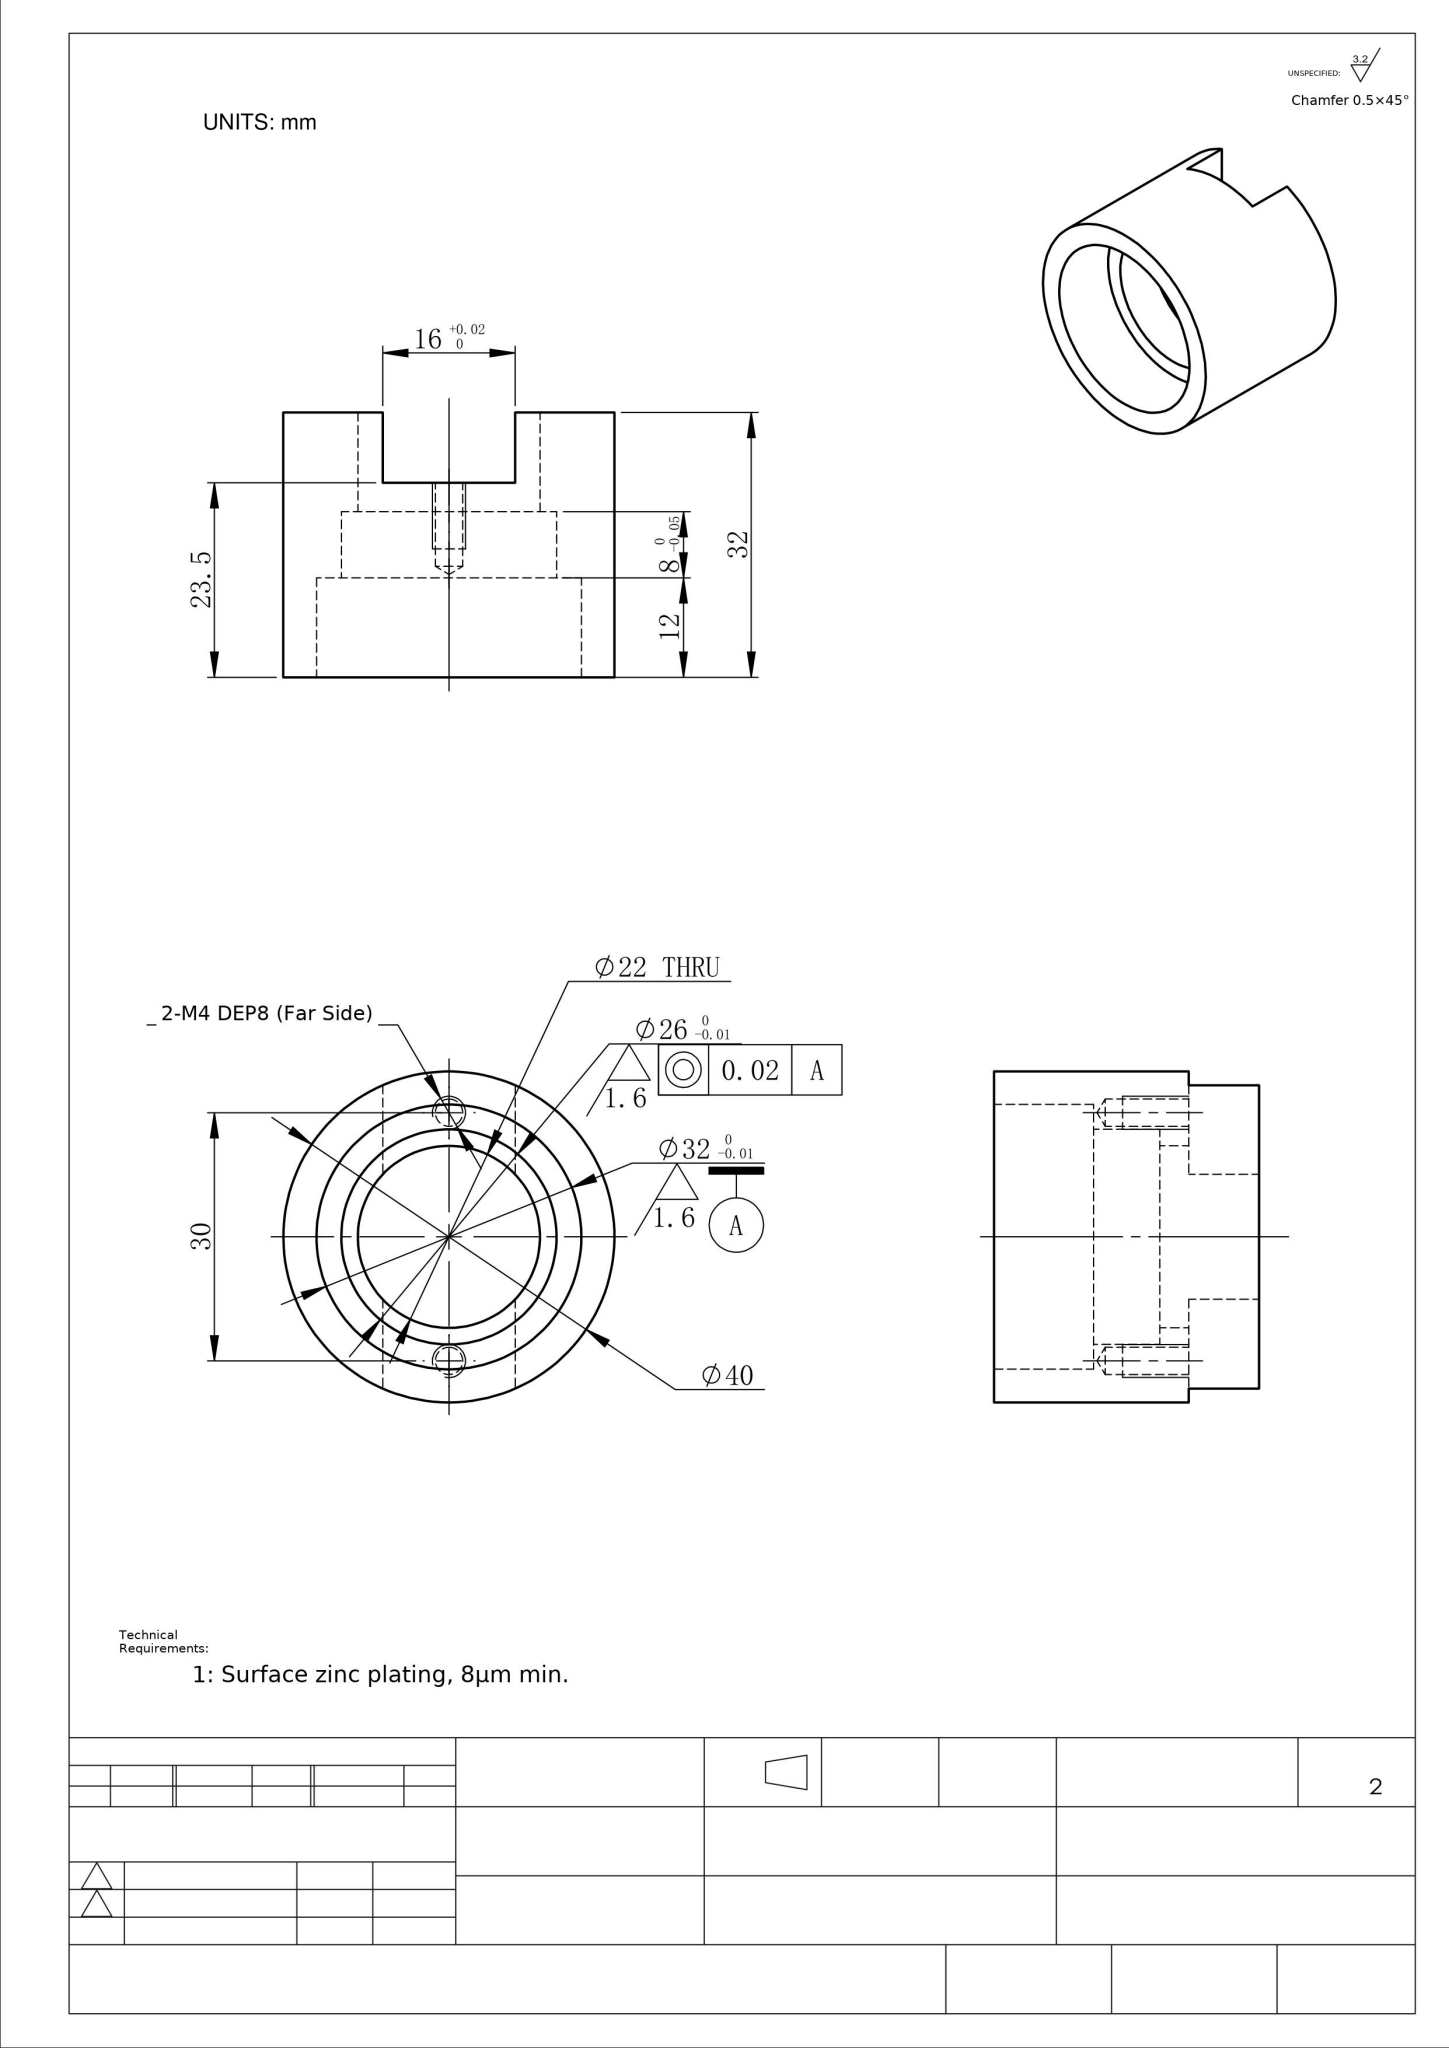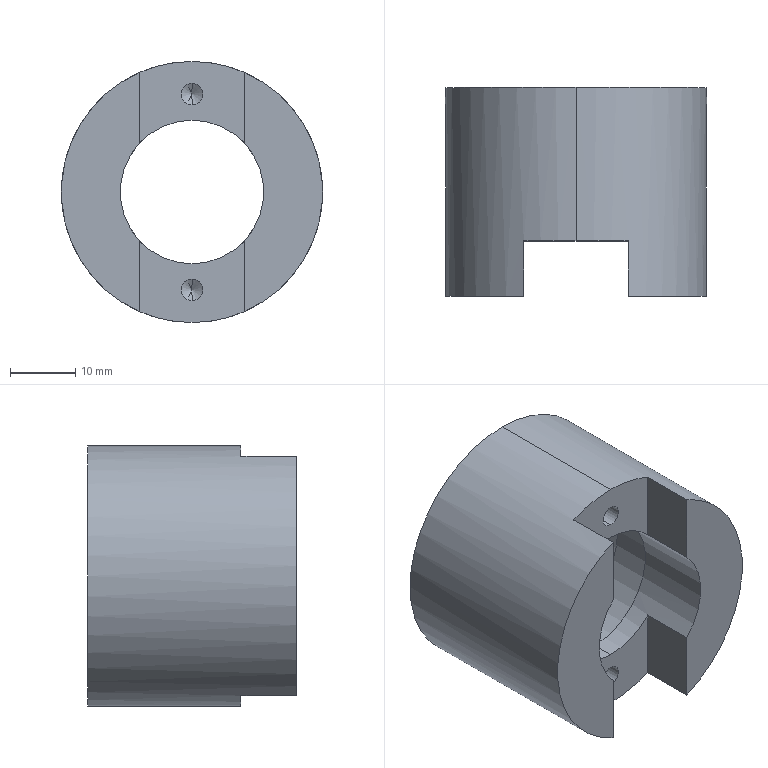Part | NX | mm | 1 solid | 27 faces | box 40 x 32 x 40 mm | volume 18985 mm3 | cylinder 12 | plane 11 | cone 4 | commonest cylinder face diameters 3.3 x4 22 x2 26 x2 32 x2 40 x2
STEP:
#1=COLOUR_RGB('',0.7961,0.8235,0.9373);
#2=FILL_AREA_STYLE_COLOUR('',#1);
#3=FILL_AREA_STYLE('',(#2));
#4=SURFACE_STYLE_FILL_AREA(#3);
#5=SURFACE_SIDE_STYLE('',(#4));
#6=SURFACE_STYLE_USAGE(.BOTH.,#5);
#7=PRESENTATION_STYLE_ASSIGNMENT((#6));
#8=CARTESIAN_POINT('',(0.,18.6,16.65));
#9=VERTEX_POINT('',#8);
#10=CARTESIAN_POINT('',(0.,18.6,13.35));
#11=VERTEX_POINT('',#10);
#12=CARTESIAN_POINT('',(0.,18.6,15.));
#13=DIRECTION('',(0.,-1.,0.));
#14=DIRECTION('',(0.,0.,-1.));
#15=AXIS2_PLACEMENT_3D('',#12,#13,#14);
#16=CIRCLE('',#15,1.65);
#17=EDGE_CURVE('',#9,#11,#16,.T.);
#18=ORIENTED_EDGE('',*,*,#17,.F.);
#19=CARTESIAN_POINT('',(0.,8.5,16.65));
#20=VERTEX_POINT('',#19);
#21=CARTESIAN_POINT('',(0.,8.5,16.65));
#22=DIRECTION('',(0.,-1.,0.));
#23=VECTOR('',#22,1000.);
#24=LINE('',#21,#23);
#25=EDGE_CURVE('',#9,#20,#24,.T.);
#26=ORIENTED_EDGE('',*,*,#25,.T.);
#27=CARTESIAN_POINT('',(0.,8.5,13.35));
#28=VERTEX_POINT('',#27);
#29=CARTESIAN_POINT('',(0.,8.5,15.));
#30=DIRECTION('',(0.,-1.,0.));
#31=DIRECTION('',(0.,0.,-1.));
#32=AXIS2_PLACEMENT_3D('',#29,#30,#31);
#33=CIRCLE('',#32,1.65);
#34=EDGE_CURVE('',#20,#28,#33,.T.);
#35=ORIENTED_EDGE('',*,*,#34,.T.);
#36=CARTESIAN_POINT('',(0.,8.5,13.35));
#37=DIRECTION('',(0.,-1.,0.));
#38=VECTOR('',#37,1000.);
#39=LINE('',#36,#38);
#40=EDGE_CURVE('',#11,#28,#39,.T.);
#41=ORIENTED_EDGE('',*,*,#40,.F.);
#42=EDGE_LOOP('',(#18,#26,#35,#41));
#43=FACE_OUTER_BOUND('',#42,.T.);
#44=CARTESIAN_POINT('',(0.,8.5,15.));
#45=DIRECTION('',(0.,-1.,0.));
#46=DIRECTION('',(0.,0.,-1.));
#47=AXIS2_PLACEMENT_3D('',#44,#45,#46);
#48=CYLINDRICAL_SURFACE('',#47,1.65);
#49=ADVANCED_FACE('',(#43),#48,.F.);
#50=STYLED_ITEM('',(#7),#49);
#51=(LENGTH_UNIT()NAMED_UNIT(*)SI_UNIT(.MILLI.,.METRE.));
#52=UNCERTAINTY_MEASURE_WITH_UNIT(LENGTH_MEASURE(0.00001),#51,'','');
#53=(NAMED_UNIT(*)PLANE_ANGLE_UNIT()SI_UNIT($,.RADIAN.));
#54=(NAMED_UNIT(*)SI_UNIT($,.STERADIAN.)SOLID_ANGLE_UNIT());
#55=(GEOMETRIC_REPRESENTATION_CONTEXT(3)GLOBAL_UNCERTAINTY_ASSIGNED_CONTEXT((#52))GLOBAL_UNIT_ASSIGNED_CONTEXT((#51,#53,#54))REPRESENTATION_CONTEXT('',''));
#56=MECHANICAL_DESIGN_GEOMETRIC_PRESENTATION_REPRESENTATION('',(#50),#55);
#57=COLOUR_RGB('',0.7961,0.8235,0.9373);
#58=FILL_AREA_STYLE_COLOUR('',#57);
#59=FILL_AREA_STYLE('',(#58));
#60=SURFACE_STYLE_FILL_AREA(#59);
#61=SURFACE_SIDE_STYLE('',(#60));
#62=SURFACE_STYLE_USAGE(.BOTH.,#61);
#63=PRESENTATION_STYLE_ASSIGNMENT((#62));
#64=CARTESIAN_POINT('',(-0.,19.591,15.));
#65=VERTEX_POINT('',#64);
#66=CARTESIAN_POINT('',(0.,18.6,13.35));
#67=DIRECTION('',(0.,-0.515,-0.8572));
#68=VECTOR('',#67,1000.);
#69=LINE('',#66,#68);
#70=EDGE_CURVE('',#65,#11,#69,.T.);
#71=ORIENTED_EDGE('',*,*,#70,.F.);
#72=CARTESIAN_POINT('',(0.,18.6,16.65));
#73=DIRECTION('',(0.,-0.515,0.8572));
#74=VECTOR('',#73,1000.);
#75=LINE('',#72,#74);
#76=EDGE_CURVE('',#65,#9,#75,.T.);
#77=ORIENTED_EDGE('',*,*,#76,.T.);
#78=ORIENTED_EDGE('',*,*,#17,.T.);
#79=EDGE_LOOP('',(#71,#77,#78));
#80=FACE_OUTER_BOUND('',#79,.T.);
#81=CARTESIAN_POINT('',(0.,18.6,15.));
#82=DIRECTION('',(0.,-1.,0.));
#83=DIRECTION('',(0.,0.,-1.));
#84=AXIS2_PLACEMENT_3D('',#81,#82,#83);
#85=CONICAL_SURFACE('',#84,1.65,1.03);
#86=ADVANCED_FACE('',(#80),#85,.F.);
#87=CARTESIAN_POINT('',(-0.,19.591,-15.));
#88=VERTEX_POINT('',#87);
#89=CARTESIAN_POINT('',(0.,18.6,-16.65));
#90=VERTEX_POINT('',#89);
#91=CARTESIAN_POINT('',(0.,18.6,-16.65));
#92=DIRECTION('',(0.,-0.515,-0.8572));
#93=VECTOR('',#92,1000.);
#94=LINE('',#91,#93);
#95=EDGE_CURVE('',#88,#90,#94,.T.);
#96=ORIENTED_EDGE('',*,*,#95,.F.);
#97=CARTESIAN_POINT('',(0.,18.6,-13.35));
#98=VERTEX_POINT('',#97);
#99=CARTESIAN_POINT('',(0.,18.6,-13.35));
#100=DIRECTION('',(0.,-0.515,0.8572));
#101=VECTOR('',#100,1000.);
#102=LINE('',#99,#101);
#103=EDGE_CURVE('',#88,#98,#102,.T.);
#104=ORIENTED_EDGE('',*,*,#103,.T.);
#105=CARTESIAN_POINT('',(0.,18.6,-15.));
#106=DIRECTION('',(0.,-1.,0.));
#107=DIRECTION('',(0.,0.,-1.));
#108=AXIS2_PLACEMENT_3D('',#105,#106,#107);
#109=CIRCLE('',#108,1.65);
#110=EDGE_CURVE('',#98,#90,#109,.T.);
#111=ORIENTED_EDGE('',*,*,#110,.T.);
#112=EDGE_LOOP('',(#96,#104,#111));
#113=FACE_OUTER_BOUND('',#112,.T.);
#114=CARTESIAN_POINT('',(0.,18.6,-15.));
#115=DIRECTION('',(0.,-1.,0.));
#116=DIRECTION('',(0.,0.,-1.));
#117=AXIS2_PLACEMENT_3D('',#114,#115,#116);
#118=CONICAL_SURFACE('',#117,1.65,1.03);
#119=ADVANCED_FACE('',(#113),#118,.F.);
#120=ORIENTED_EDGE('',*,*,#110,.F.);
#121=CARTESIAN_POINT('',(0.,8.5,-13.35));
#122=VERTEX_POINT('',#121);
#123=CARTESIAN_POINT('',(0.,8.5,-13.35));
#124=DIRECTION('',(0.,-1.,0.));
#125=VECTOR('',#124,1000.);
#126=LINE('',#123,#125);
#127=EDGE_CURVE('',#98,#122,#126,.T.);
#128=ORIENTED_EDGE('',*,*,#127,.T.);
#129=CARTESIAN_POINT('',(0.,8.5,-16.65));
#130=VERTEX_POINT('',#129);
#131=CARTESIAN_POINT('',(0.,8.5,-15.));
#132=DIRECTION('',(0.,-1.,0.));
#133=DIRECTION('',(0.,0.,-1.));
#134=AXIS2_PLACEMENT_3D('',#131,#132,#133);
#135=CIRCLE('',#134,1.65);
#136=EDGE_CURVE('',#122,#130,#135,.T.);
#137=ORIENTED_EDGE('',*,*,#136,.T.);
#138=CARTESIAN_POINT('',(0.,8.5,-16.65));
#139=DIRECTION('',(0.,-1.,0.));
#140=VECTOR('',#139,1000.);
#141=LINE('',#138,#140);
#142=EDGE_CURVE('',#90,#130,#141,.T.);
#143=ORIENTED_EDGE('',*,*,#142,.F.);
#144=EDGE_LOOP('',(#120,#128,#137,#143));
#145=FACE_OUTER_BOUND('',#144,.T.);
#146=CARTESIAN_POINT('',(0.,8.5,-15.));
#147=DIRECTION('',(0.,-1.,0.));
#148=DIRECTION('',(0.,0.,-1.));
#149=AXIS2_PLACEMENT_3D('',#146,#147,#148);
#150=CYLINDRICAL_SURFACE('',#149,1.65);
#151=ADVANCED_FACE('',(#145),#150,.F.);
#152=CARTESIAN_POINT('',(-8.,8.5,-7.55));
#153=VERTEX_POINT('',#152);
#154=CARTESIAN_POINT('',(0.,8.5,-11.));
#155=VERTEX_POINT('',#154);
#156=CARTESIAN_POINT('',(0.,8.5,0.));
#157=DIRECTION('',(0.,-1.,0.));
#158=DIRECTION('',(0.,0.,1.));
#159=AXIS2_PLACEMENT_3D('',#156,#157,#158);
#160=CIRCLE('',#159,11.);
#161=EDGE_CURVE('',#153,#155,#160,.T.);
#162=ORIENTED_EDGE('',*,*,#161,.T.);
#163=CARTESIAN_POINT('',(0.,12.,-11.));
#164=VERTEX_POINT('',#163);
#165=CARTESIAN_POINT('',(0.,88.583,-11.));
#166=DIRECTION('',(0.,1.,0.));
#167=VECTOR('',#166,1000.);
#168=LINE('',#165,#167);
#169=EDGE_CURVE('',#155,#164,#168,.T.);
#170=ORIENTED_EDGE('',*,*,#169,.T.);
#171=CARTESIAN_POINT('',(0.,12.,11.));
#172=VERTEX_POINT('',#171);
#173=CARTESIAN_POINT('',(0.,12.,0.));
#174=DIRECTION('',(0.,1.,0.));
#175=DIRECTION('',(0.,0.,1.));
#176=AXIS2_PLACEMENT_3D('',#173,#174,#175);
#177=CIRCLE('',#176,11.);
#178=EDGE_CURVE('',#164,#172,#177,.T.);
#179=ORIENTED_EDGE('',*,*,#178,.T.);
#180=CARTESIAN_POINT('',(0.,8.5,11.));
#181=VERTEX_POINT('',#180);
#182=CARTESIAN_POINT('',(0.,88.583,11.));
#183=DIRECTION('',(0.,1.,0.));
#184=VECTOR('',#183,1000.);
#185=LINE('',#182,#184);
#186=EDGE_CURVE('',#181,#172,#185,.T.);
#187=ORIENTED_EDGE('',*,*,#186,.F.);
#188=CARTESIAN_POINT('',(-8.,8.5,7.55));
#189=VERTEX_POINT('',#188);
#190=CARTESIAN_POINT('',(0.,8.5,0.));
#191=DIRECTION('',(0.,-1.,0.));
#192=DIRECTION('',(0.,0.,1.));
#193=AXIS2_PLACEMENT_3D('',#190,#191,#192);
#194=CIRCLE('',#193,11.);
#195=EDGE_CURVE('',#181,#189,#194,.T.);
#196=ORIENTED_EDGE('',*,*,#195,.T.);
#197=CARTESIAN_POINT('',(-8.,0.,7.55));
#198=VERTEX_POINT('',#197);
#199=CARTESIAN_POINT('',(-8.,88.583,7.55));
#200=DIRECTION('',(0.,-1.,0.));
#201=VECTOR('',#200,1000.);
#202=LINE('',#199,#201);
#203=EDGE_CURVE('',#189,#198,#202,.T.);
#204=ORIENTED_EDGE('',*,*,#203,.T.);
#205=CARTESIAN_POINT('',(-8.,0.,-7.55));
#206=VERTEX_POINT('',#205);
#207=CARTESIAN_POINT('',(0.,0.,0.));
#208=DIRECTION('',(0.,1.,0.));
#209=DIRECTION('',(0.,0.,1.));
#210=AXIS2_PLACEMENT_3D('',#207,#208,#209);
#211=CIRCLE('',#210,11.);
#212=EDGE_CURVE('',#206,#198,#211,.T.);
#213=ORIENTED_EDGE('',*,*,#212,.F.);
#214=CARTESIAN_POINT('',(-8.,88.583,-7.55));
#215=DIRECTION('',(0.,1.,0.));
#216=VECTOR('',#215,1000.);
#217=LINE('',#214,#216);
#218=EDGE_CURVE('',#206,#153,#217,.T.);
#219=ORIENTED_EDGE('',*,*,#218,.T.);
#220=EDGE_LOOP('',(#162,#170,#179,#187,#196,#204,#213,#219));
#221=FACE_OUTER_BOUND('',#220,.T.);
#222=CARTESIAN_POINT('',(0.,88.583,0.));
#223=DIRECTION('',(0.,1.,0.));
#224=DIRECTION('',(0.,0.,1.));
#225=AXIS2_PLACEMENT_3D('',#222,#223,#224);
#226=CYLINDRICAL_SURFACE('',#225,11.);
#227=ADVANCED_FACE('',(#221),#226,.F.);
#228=CARTESIAN_POINT('',(0.,12.,-13.));
#229=VERTEX_POINT('',#228);
#230=CARTESIAN_POINT('',(0.,12.,13.));
#231=VERTEX_POINT('',#230);
#232=CARTESIAN_POINT('',(0.,12.,0.));
#233=DIRECTION('',(0.,1.,0.));
#234=DIRECTION('',(0.,0.,1.));
#235=AXIS2_PLACEMENT_3D('',#232,#233,#234);
#236=CIRCLE('',#235,13.);
#237=EDGE_CURVE('',#229,#231,#236,.T.);
#238=ORIENTED_EDGE('',*,*,#237,.F.);
#239=CARTESIAN_POINT('',(0.,20.,-13.));
#240=VERTEX_POINT('',#239);
#241=CARTESIAN_POINT('',(0.,88.583,-13.));
#242=DIRECTION('',(0.,1.,0.));
#243=VECTOR('',#242,1000.);
#244=LINE('',#241,#243);
#245=EDGE_CURVE('',#229,#240,#244,.T.);
#246=ORIENTED_EDGE('',*,*,#245,.T.);
#247=CARTESIAN_POINT('',(0.,20.,13.));
#248=VERTEX_POINT('',#247);
#249=CARTESIAN_POINT('',(0.,20.,0.));
#250=DIRECTION('',(0.,1.,0.));
#251=DIRECTION('',(0.,0.,1.));
#252=AXIS2_PLACEMENT_3D('',#249,#250,#251);
#253=CIRCLE('',#252,13.);
#254=EDGE_CURVE('',#240,#248,#253,.T.);
#255=ORIENTED_EDGE('',*,*,#254,.T.);
#256=CARTESIAN_POINT('',(0.,88.583,13.));
#257=DIRECTION('',(0.,1.,0.));
#258=VECTOR('',#257,1000.);
#259=LINE('',#256,#258);
#260=EDGE_CURVE('',#231,#248,#259,.T.);
#261=ORIENTED_EDGE('',*,*,#260,.F.);
#262=EDGE_LOOP('',(#238,#246,#255,#261));
#263=FACE_OUTER_BOUND('',#262,.T.);
#264=CARTESIAN_POINT('',(0.,88.583,0.));
#265=DIRECTION('',(0.,1.,0.));
#266=DIRECTION('',(0.,0.,1.));
#267=AXIS2_PLACEMENT_3D('',#264,#265,#266);
#268=CYLINDRICAL_SURFACE('',#267,13.);
#269=ADVANCED_FACE('',(#263),#268,.F.);
#270=CARTESIAN_POINT('',(0.,20.,-16.));
#271=VERTEX_POINT('',#270);
#272=CARTESIAN_POINT('',(0.,20.,16.));
#273=VERTEX_POINT('',#272);
#274=CARTESIAN_POINT('',(0.,20.,0.));
#275=DIRECTION('',(0.,1.,0.));
#276=DIRECTION('',(0.,0.,1.));
#277=AXIS2_PLACEMENT_3D('',#274,#275,#276);
#278=CIRCLE('',#277,16.);
#279=EDGE_CURVE('',#271,#273,#278,.T.);
#280=ORIENTED_EDGE('',*,*,#279,.F.);
#281=CARTESIAN_POINT('',(0.,32.,-16.));
#282=VERTEX_POINT('',#281);
#283=CARTESIAN_POINT('',(0.,88.583,-16.));
#284=DIRECTION('',(0.,1.,0.));
#285=VECTOR('',#284,1000.);
#286=LINE('',#283,#285);
#287=EDGE_CURVE('',#271,#282,#286,.T.);
#288=ORIENTED_EDGE('',*,*,#287,.T.);
#289=CARTESIAN_POINT('',(0.,32.,16.));
#290=VERTEX_POINT('',#289);
#291=CARTESIAN_POINT('',(0.,32.,0.));
#292=DIRECTION('',(0.,1.,0.));
#293=DIRECTION('',(0.,0.,1.));
#294=AXIS2_PLACEMENT_3D('',#291,#292,#293);
#295=CIRCLE('',#294,16.);
#296=EDGE_CURVE('',#282,#290,#295,.T.);
#297=ORIENTED_EDGE('',*,*,#296,.T.);
#298=CARTESIAN_POINT('',(0.,88.583,16.));
#299=DIRECTION('',(0.,1.,0.));
#300=VECTOR('',#299,1000.);
#301=LINE('',#298,#300);
#302=EDGE_CURVE('',#273,#290,#301,.T.);
#303=ORIENTED_EDGE('',*,*,#302,.F.);
#304=EDGE_LOOP('',(#280,#288,#297,#303));
#305=FACE_OUTER_BOUND('',#304,.T.);
#306=CARTESIAN_POINT('',(0.,88.583,0.));
#307=DIRECTION('',(0.,1.,0.));
#308=DIRECTION('',(0.,0.,1.));
#309=AXIS2_PLACEMENT_3D('',#306,#307,#308);
#310=CYLINDRICAL_SURFACE('',#309,16.);
#311=ADVANCED_FACE('',(#305),#310,.F.);
#312=CARTESIAN_POINT('',(8.,8.5,-18.33));
#313=VERTEX_POINT('',#312);
#314=CARTESIAN_POINT('',(0.,8.5,-20.));
#315=VERTEX_POINT('',#314);
#316=CARTESIAN_POINT('',(0.,8.5,0.));
#317=DIRECTION('',(0.,1.,0.));
#318=DIRECTION('',(0.,0.,1.));
#319=AXIS2_PLACEMENT_3D('',#316,#317,#318);
#320=CIRCLE('',#319,20.);
#321=EDGE_CURVE('',#313,#315,#320,.T.);
#322=ORIENTED_EDGE('',*,*,#321,.T.);
#323=CARTESIAN_POINT('',(0.,32.,-20.));
#324=VERTEX_POINT('',#323);
#325=CARTESIAN_POINT('',(0.,88.583,-20.));
#326=DIRECTION('',(0.,1.,0.));
#327=VECTOR('',#326,1000.);
#328=LINE('',#325,#327);
#329=EDGE_CURVE('',#315,#324,#328,.T.);
#330=ORIENTED_EDGE('',*,*,#329,.T.);
#331=CARTESIAN_POINT('',(0.,32.,20.));
#332=VERTEX_POINT('',#331);
#333=CARTESIAN_POINT('',(0.,32.,0.));
#334=DIRECTION('',(0.,1.,0.));
#335=DIRECTION('',(0.,0.,1.));
#336=AXIS2_PLACEMENT_3D('',#333,#334,#335);
#337=CIRCLE('',#336,20.);
#338=EDGE_CURVE('',#332,#324,#337,.T.);
#339=ORIENTED_EDGE('',*,*,#338,.F.);
#340=CARTESIAN_POINT('',(0.,8.5,20.));
#341=VERTEX_POINT('',#340);
#342=CARTESIAN_POINT('',(0.,88.583,20.));
#343=DIRECTION('',(0.,1.,0.));
#344=VECTOR('',#343,1000.);
#345=LINE('',#342,#344);
#346=EDGE_CURVE('',#341,#332,#345,.T.);
#347=ORIENTED_EDGE('',*,*,#346,.F.);
#348=CARTESIAN_POINT('',(8.,8.5,18.33));
#349=VERTEX_POINT('',#348);
#350=CARTESIAN_POINT('',(0.,8.5,0.));
#351=DIRECTION('',(0.,1.,0.));
#352=DIRECTION('',(0.,0.,1.));
#353=AXIS2_PLACEMENT_3D('',#350,#351,#352);
#354=CIRCLE('',#353,20.);
#355=EDGE_CURVE('',#341,#349,#354,.T.);
#356=ORIENTED_EDGE('',*,*,#355,.T.);
#357=CARTESIAN_POINT('',(8.,0.,18.33));
#358=VERTEX_POINT('',#357);
#359=CARTESIAN_POINT('',(8.,88.583,18.33));
#360=DIRECTION('',(0.,-1.,0.));
#361=VECTOR('',#360,1000.);
#362=LINE('',#359,#361);
#363=EDGE_CURVE('',#349,#358,#362,.T.);
#364=ORIENTED_EDGE('',*,*,#363,.T.);
#365=CARTESIAN_POINT('',(8.,0.,-18.33));
#366=VERTEX_POINT('',#365);
#367=CARTESIAN_POINT('',(0.,0.,0.));
#368=DIRECTION('',(0.,1.,0.));
#369=DIRECTION('',(0.,0.,1.));
#370=AXIS2_PLACEMENT_3D('',#367,#368,#369);
#371=CIRCLE('',#370,20.);
#372=EDGE_CURVE('',#358,#366,#371,.T.);
#373=ORIENTED_EDGE('',*,*,#372,.T.);
#374=CARTESIAN_POINT('',(8.,88.583,-18.33));
#375=DIRECTION('',(0.,1.,0.));
#376=VECTOR('',#375,1000.);
#377=LINE('',#374,#376);
#378=EDGE_CURVE('',#366,#313,#377,.T.);
#379=ORIENTED_EDGE('',*,*,#378,.T.);
#380=EDGE_LOOP('',(#322,#330,#339,#347,#356,#364,#373,#379));
#381=FACE_OUTER_BOUND('',#380,.T.);
#382=CARTESIAN_POINT('',(0.,88.583,0.));
#383=DIRECTION('',(0.,1.,0.));
#384=DIRECTION('',(0.,0.,1.));
#385=AXIS2_PLACEMENT_3D('',#382,#383,#384);
#386=CYLINDRICAL_SURFACE('',#385,20.);
#387=ADVANCED_FACE('',(#381),#386,.T.);
#388=CARTESIAN_POINT('',(-8.,0.,-18.33));
#389=VERTEX_POINT('',#388);
#390=CARTESIAN_POINT('',(-8.,0.,18.33));
#391=VERTEX_POINT('',#390);
#392=CARTESIAN_POINT('',(0.,0.,0.));
#393=DIRECTION('',(0.,1.,0.));
#394=DIRECTION('',(0.,0.,1.));
#395=AXIS2_PLACEMENT_3D('',#392,#393,#394);
#396=CIRCLE('',#395,20.);
#397=EDGE_CURVE('',#389,#391,#396,.T.);
#398=ORIENTED_EDGE('',*,*,#397,.F.);
#399=CARTESIAN_POINT('',(-8.,-0.,0.));
#400=DIRECTION('',(0.,0.,1.));
#401=VECTOR('',#400,1000.);
#402=LINE('',#399,#401);
#403=EDGE_CURVE('',#389,#206,#402,.T.);
#404=ORIENTED_EDGE('',*,*,#403,.T.);
#405=ORIENTED_EDGE('',*,*,#212,.T.);
#406=CARTESIAN_POINT('',(-8.,-0.,0.));
#407=DIRECTION('',(0.,0.,1.));
#408=VECTOR('',#407,1000.);
#409=LINE('',#406,#408);
#410=EDGE_CURVE('',#198,#391,#409,.T.);
#411=ORIENTED_EDGE('',*,*,#410,.T.);
#412=EDGE_LOOP('',(#398,#404,#405,#411));
#413=FACE_OUTER_BOUND('',#412,.T.);
#414=CARTESIAN_POINT('',(20.,-0.,0.));
#415=DIRECTION('',(0.,1.,0.));
#416=DIRECTION('',(0.,0.,1.));
#417=AXIS2_PLACEMENT_3D('',#414,#415,#416);
#418=PLANE('',#417);
#419=ADVANCED_FACE('',(#413),#418,.F.);
#420=ORIENTED_EDGE('',*,*,#329,.F.);
#421=CARTESIAN_POINT('',(-8.,8.5,-18.33));
#422=VERTEX_POINT('',#421);
#423=CARTESIAN_POINT('',(0.,8.5,0.));
#424=DIRECTION('',(0.,1.,0.));
#425=DIRECTION('',(0.,0.,1.));
#426=AXIS2_PLACEMENT_3D('',#423,#424,#425);
#427=CIRCLE('',#426,20.);
#428=EDGE_CURVE('',#315,#422,#427,.T.);
#429=ORIENTED_EDGE('',*,*,#428,.T.);
#430=CARTESIAN_POINT('',(-8.,88.583,-18.33));
#431=DIRECTION('',(0.,-1.,0.));
#432=VECTOR('',#431,1000.);
#433=LINE('',#430,#432);
#434=EDGE_CURVE('',#422,#389,#433,.T.);
#435=ORIENTED_EDGE('',*,*,#434,.T.);
#436=ORIENTED_EDGE('',*,*,#397,.T.);
#437=CARTESIAN_POINT('',(-8.,8.5,18.33));
#438=VERTEX_POINT('',#437);
#439=CARTESIAN_POINT('',(-8.,88.583,18.33));
#440=DIRECTION('',(0.,1.,0.));
#441=VECTOR('',#440,1000.);
#442=LINE('',#439,#441);
#443=EDGE_CURVE('',#391,#438,#442,.T.);
#444=ORIENTED_EDGE('',*,*,#443,.T.);
#445=CARTESIAN_POINT('',(0.,8.5,0.));
#446=DIRECTION('',(0.,1.,0.));
#447=DIRECTION('',(0.,0.,1.));
#448=AXIS2_PLACEMENT_3D('',#445,#446,#447);
#449=CIRCLE('',#448,20.);
#450=EDGE_CURVE('',#438,#341,#449,.T.);
#451=ORIENTED_EDGE('',*,*,#450,.T.);
#452=ORIENTED_EDGE('',*,*,#346,.T.);
#453=CARTESIAN_POINT('',(0.,32.,0.));
#454=DIRECTION('',(0.,1.,0.));
#455=DIRECTION('',(0.,0.,1.));
#456=AXIS2_PLACEMENT_3D('',#453,#454,#455);
#457=CIRCLE('',#456,20.);
#458=EDGE_CURVE('',#324,#332,#457,.T.);
#459=ORIENTED_EDGE('',*,*,#458,.F.);
#460=EDGE_LOOP('',(#420,#429,#435,#436,#444,#451,#452,#459));
#461=FACE_OUTER_BOUND('',#460,.T.);
#462=CARTESIAN_POINT('',(0.,88.583,0.));
#463=DIRECTION('',(0.,1.,0.));
#464=DIRECTION('',(0.,0.,1.));
#465=AXIS2_PLACEMENT_3D('',#462,#463,#464);
#466=CYLINDRICAL_SURFACE('',#465,20.);
#467=ADVANCED_FACE('',(#461),#466,.T.);
#468=CARTESIAN_POINT('',(0.,32.,0.));
#469=DIRECTION('',(0.,1.,0.));
#470=DIRECTION('',(0.,0.,1.));
#471=AXIS2_PLACEMENT_3D('',#468,#469,#470);
#472=CIRCLE('',#471,16.);
#473=EDGE_CURVE('',#290,#282,#472,.T.);
#474=ORIENTED_EDGE('',*,*,#473,.F.);
#475=ORIENTED_EDGE('',*,*,#296,.F.);
#476=EDGE_LOOP('',(#474,#475));
#477=FACE_BOUND('',#476,.T.);
#478=ORIENTED_EDGE('',*,*,#338,.T.);
#479=ORIENTED_EDGE('',*,*,#458,.T.);
#480=EDGE_LOOP('',(#478,#479));
#481=FACE_OUTER_BOUND('',#480,.T.);
#482=CARTESIAN_POINT('',(20.,32.,0.));
#483=DIRECTION('',(0.,-1.,0.));
#484=DIRECTION('',(0.,0.,-1.));
#485=AXIS2_PLACEMENT_3D('',#482,#483,#484);
#486=PLANE('',#485);
#487=ADVANCED_FACE('',(#477,#481),#486,.F.);
#488=ORIENTED_EDGE('',*,*,#287,.F.);
#489=CARTESIAN_POINT('',(0.,20.,0.));
#490=DIRECTION('',(0.,1.,0.));
#491=DIRECTION('',(0.,0.,1.));
#492=AXIS2_PLACEMENT_3D('',#489,#490,#491);
#493=CIRCLE('',#492,16.);
#494=EDGE_CURVE('',#273,#271,#493,.T.);
#495=ORIENTED_EDGE('',*,*,#494,.F.);
#496=ORIENTED_EDGE('',*,*,#302,.T.);
#497=ORIENTED_EDGE('',*,*,#473,.T.);
#498=EDGE_LOOP('',(#488,#495,#496,#497));
#499=FACE_OUTER_BOUND('',#498,.T.);
#500=CARTESIAN_POINT('',(0.,88.583,0.));
#501=DIRECTION('',(0.,1.,0.));
#502=DIRECTION('',(0.,0.,1.));
#503=AXIS2_PLACEMENT_3D('',#500,#501,#502);
#504=CYLINDRICAL_SURFACE('',#503,16.);
#505=ADVANCED_FACE('',(#499),#504,.F.);
#506=CARTESIAN_POINT('',(0.,20.,0.));
#507=DIRECTION('',(0.,1.,0.));
#508=DIRECTION('',(0.,0.,1.));
#509=AXIS2_PLACEMENT_3D('',#506,#507,#508);
#510=CIRCLE('',#509,13.);
#511=EDGE_CURVE('',#248,#240,#510,.T.);
#512=ORIENTED_EDGE('',*,*,#511,.F.);
#513=ORIENTED_EDGE('',*,*,#254,.F.);
#514=EDGE_LOOP('',(#512,#513));
#515=FACE_BOUND('',#514,.T.);
#516=ORIENTED_EDGE('',*,*,#494,.T.);
#517=ORIENTED_EDGE('',*,*,#279,.T.);
#518=EDGE_LOOP('',(#516,#517));
#519=FACE_OUTER_BOUND('',#518,.T.);
#520=CARTESIAN_POINT('',(16.,20.,0.));
#521=DIRECTION('',(0.,-1.,0.));
#522=DIRECTION('',(0.,0.,-1.));
#523=AXIS2_PLACEMENT_3D('',#520,#521,#522);
#524=PLANE('',#523);
#525=ADVANCED_FACE('',(#515,#519),#524,.F.);
#526=ORIENTED_EDGE('',*,*,#245,.F.);
#527=CARTESIAN_POINT('',(0.,12.,0.));
#528=DIRECTION('',(0.,1.,0.));
#529=DIRECTION('',(0.,0.,1.));
#530=AXIS2_PLACEMENT_3D('',#527,#528,#529);
#531=CIRCLE('',#530,13.);
#532=EDGE_CURVE('',#231,#229,#531,.T.);
#533=ORIENTED_EDGE('',*,*,#532,.F.);
#534=ORIENTED_EDGE('',*,*,#260,.T.);
#535=ORIENTED_EDGE('',*,*,#511,.T.);
#536=EDGE_LOOP('',(#526,#533,#534,#535));
#537=FACE_OUTER_BOUND('',#536,.T.);
#538=CARTESIAN_POINT('',(0.,88.583,0.));
#539=DIRECTION('',(0.,1.,0.));
#540=DIRECTION('',(0.,0.,1.));
#541=AXIS2_PLACEMENT_3D('',#538,#539,#540);
#542=CYLINDRICAL_SURFACE('',#541,13.);
#543=ADVANCED_FACE('',(#537),#542,.F.);
#544=CARTESIAN_POINT('',(0.,12.,0.));
#545=DIRECTION('',(0.,1.,0.));
#546=DIRECTION('',(0.,0.,1.));
#547=AXIS2_PLACEMENT_3D('',#544,#545,#546);
#548=CIRCLE('',#547,11.);
#549=EDGE_CURVE('',#172,#164,#548,.T.);
#550=ORIENTED_EDGE('',*,*,#549,.F.);
#551=ORIENTED_EDGE('',*,*,#178,.F.);
#552=EDGE_LOOP('',(#550,#551));
#553=FACE_BOUND('',#552,.T.);
#554=ORIENTED_EDGE('',*,*,#532,.T.);
#555=ORIENTED_EDGE('',*,*,#237,.T.);
#556=EDGE_LOOP('',(#554,#555));
#557=FACE_OUTER_BOUND('',#556,.T.);
#558=CARTESIAN_POINT('',(13.,12.,0.));
#559=DIRECTION('',(0.,-1.,0.));
#560=DIRECTION('',(0.,0.,-1.));
#561=AXIS2_PLACEMENT_3D('',#558,#559,#560);
#562=PLANE('',#561);
#563=ADVANCED_FACE('',(#553,#557),#562,.F.);
#564=ORIENTED_EDGE('',*,*,#169,.F.);
#565=CARTESIAN_POINT('',(8.,8.5,-7.55));
#566=VERTEX_POINT('',#565);
#567=CARTESIAN_POINT('',(0.,8.5,0.));
#568=DIRECTION('',(0.,-1.,0.));
#569=DIRECTION('',(0.,0.,1.));
#570=AXIS2_PLACEMENT_3D('',#567,#568,#569);
#571=CIRCLE('',#570,11.);
#572=EDGE_CURVE('',#155,#566,#571,.T.);
#573=ORIENTED_EDGE('',*,*,#572,.T.);
#574=CARTESIAN_POINT('',(8.,0.,-7.55));
#575=VERTEX_POINT('',#574);
#576=CARTESIAN_POINT('',(8.,88.583,-7.55));
#577=DIRECTION('',(0.,-1.,0.));
#578=VECTOR('',#577,1000.);
#579=LINE('',#576,#578);
#580=EDGE_CURVE('',#566,#575,#579,.T.);
#581=ORIENTED_EDGE('',*,*,#580,.T.);
#582=CARTESIAN_POINT('',(8.,0.,7.55));
#583=VERTEX_POINT('',#582);
#584=CARTESIAN_POINT('',(0.,0.,0.));
#585=DIRECTION('',(0.,1.,0.));
#586=DIRECTION('',(0.,0.,1.));
#587=AXIS2_PLACEMENT_3D('',#584,#585,#586);
#588=CIRCLE('',#587,11.);
#589=EDGE_CURVE('',#583,#575,#588,.T.);
#590=ORIENTED_EDGE('',*,*,#589,.F.);
#591=CARTESIAN_POINT('',(8.,8.5,7.55));
#592=VERTEX_POINT('',#591);
#593=CARTESIAN_POINT('',(8.,88.583,7.55));
#594=DIRECTION('',(0.,1.,0.));
#595=VECTOR('',#594,1000.);
#596=LINE('',#593,#595);
#597=EDGE_CURVE('',#583,#592,#596,.T.);
#598=ORIENTED_EDGE('',*,*,#597,.T.);
#599=CARTESIAN_POINT('',(0.,8.5,0.));
#600=DIRECTION('',(0.,-1.,0.));
#601=DIRECTION('',(-0.,0.,1.));
#602=AXIS2_PLACEMENT_3D('',#599,#600,#601);
#603=CIRCLE('',#602,11.);
#604=EDGE_CURVE('',#592,#181,#603,.T.);
#605=ORIENTED_EDGE('',*,*,#604,.T.);
#606=ORIENTED_EDGE('',*,*,#186,.T.);
#607=ORIENTED_EDGE('',*,*,#549,.T.);
#608=EDGE_LOOP('',(#564,#573,#581,#590,#598,#605,#606,#607));
#609=FACE_OUTER_BOUND('',#608,.T.);
#610=CARTESIAN_POINT('',(0.,88.583,0.));
#611=DIRECTION('',(0.,1.,0.));
#612=DIRECTION('',(0.,0.,1.));
#613=AXIS2_PLACEMENT_3D('',#610,#611,#612);
#614=CYLINDRICAL_SURFACE('',#613,11.);
#615=ADVANCED_FACE('',(#609),#614,.F.);
#616=ORIENTED_EDGE('',*,*,#372,.F.);
#617=CARTESIAN_POINT('',(8.,-0.,0.));
#618=DIRECTION('',(0.,0.,-1.));
#619=VECTOR('',#618,1000.);
#620=LINE('',#617,#619);
#621=EDGE_CURVE('',#358,#583,#620,.T.);
#622=ORIENTED_EDGE('',*,*,#621,.T.);
#623=ORIENTED_EDGE('',*,*,#589,.T.);
#624=CARTESIAN_POINT('',(8.,-0.,0.));
#625=DIRECTION('',(0.,0.,-1.));
#626=VECTOR('',#625,1000.);
#627=LINE('',#624,#626);
#628=EDGE_CURVE('',#575,#366,#627,.T.);
#629=ORIENTED_EDGE('',*,*,#628,.T.);
#630=EDGE_LOOP('',(#616,#622,#623,#629));
#631=FACE_OUTER_BOUND('',#630,.T.);
#632=CARTESIAN_POINT('',(20.,-0.,0.));
#633=DIRECTION('',(0.,1.,0.));
#634=DIRECTION('',(0.,0.,1.));
#635=AXIS2_PLACEMENT_3D('',#632,#633,#634);
#636=PLANE('',#635);
#637=ADVANCED_FACE('',(#631),#636,.F.);
#638=CARTESIAN_POINT('',(-8.,8.5,-20.));
#639=DIRECTION('',(0.,0.,1.));
#640=VECTOR('',#639,1000.);
#641=LINE('',#638,#640);
#642=EDGE_CURVE('',#422,#153,#641,.T.);
#643=ORIENTED_EDGE('',*,*,#642,.T.);
#644=ORIENTED_EDGE('',*,*,#218,.F.);
#645=ORIENTED_EDGE('',*,*,#403,.F.);
#646=ORIENTED_EDGE('',*,*,#434,.F.);
#647=EDGE_LOOP('',(#643,#644,#645,#646));
#648=FACE_OUTER_BOUND('',#647,.T.);
#649=CARTESIAN_POINT('',(-8.,0.,-20.));
#650=DIRECTION('',(-1.,0.,0.));
#651=DIRECTION('',(0.,0.,1.));
#652=AXIS2_PLACEMENT_3D('',#649,#650,#651);
#653=PLANE('',#652);
#654=ADVANCED_FACE('',(#648),#653,.F.);
#655=ORIENTED_EDGE('',*,*,#628,.F.);
#656=ORIENTED_EDGE('',*,*,#580,.F.);
#657=CARTESIAN_POINT('',(8.,8.5,-20.));
#658=DIRECTION('',(0.,0.,1.));
#659=VECTOR('',#658,1000.);
#660=LINE('',#657,#659);
#661=EDGE_CURVE('',#313,#566,#660,.T.);
#662=ORIENTED_EDGE('',*,*,#661,.F.);
#663=ORIENTED_EDGE('',*,*,#378,.F.);
#664=EDGE_LOOP('',(#655,#656,#662,#663));
#665=FACE_OUTER_BOUND('',#664,.T.);
#666=CARTESIAN_POINT('',(8.,0.,-20.));
#667=DIRECTION('',(1.,0.,0.));
#668=DIRECTION('',(0.,0.,-1.));
#669=AXIS2_PLACEMENT_3D('',#666,#667,#668);
#670=PLANE('',#669);
#671=ADVANCED_FACE('',(#665),#670,.F.);
#672=CARTESIAN_POINT('',(0.,8.5,-15.));
#673=DIRECTION('',(0.,-1.,0.));
#674=DIRECTION('',(0.,0.,-1.));
#675=AXIS2_PLACEMENT_3D('',#672,#673,#674);
#676=CIRCLE('',#675,1.65);
#677=EDGE_CURVE('',#130,#122,#676,.T.);
#678=ORIENTED_EDGE('',*,*,#677,.F.);
#679=ORIENTED_EDGE('',*,*,#136,.F.);
#680=EDGE_LOOP('',(#678,#679));
#681=FACE_BOUND('',#680,.T.);
#682=ORIENTED_EDGE('',*,*,#661,.T.);
#683=ORIENTED_EDGE('',*,*,#572,.F.);
#684=ORIENTED_EDGE('',*,*,#161,.F.);
#685=ORIENTED_EDGE('',*,*,#642,.F.);
#686=ORIENTED_EDGE('',*,*,#428,.F.);
#687=ORIENTED_EDGE('',*,*,#321,.F.);
#688=EDGE_LOOP('',(#682,#683,#684,#685,#686,#687));
#689=FACE_OUTER_BOUND('',#688,.T.);
#690=CARTESIAN_POINT('',(-8.,8.5,-20.));
#691=DIRECTION('',(0.,1.,0.));
#692=DIRECTION('',(0.,0.,1.));
#693=AXIS2_PLACEMENT_3D('',#690,#691,#692);
#694=PLANE('',#693);
#695=ADVANCED_FACE('',(#681,#689),#694,.F.);
#696=CARTESIAN_POINT('',(0.,8.5,15.));
#697=DIRECTION('',(0.,-1.,0.));
#698=DIRECTION('',(0.,0.,-1.));
#699=AXIS2_PLACEMENT_3D('',#696,#697,#698);
#700=CIRCLE('',#699,1.65);
#701=EDGE_CURVE('',#28,#20,#700,.T.);
#702=ORIENTED_EDGE('',*,*,#701,.F.);
#703=ORIENTED_EDGE('',*,*,#34,.F.);
#704=EDGE_LOOP('',(#702,#703));
#705=FACE_BOUND('',#704,.T.);
#706=ORIENTED_EDGE('',*,*,#450,.F.);
#707=CARTESIAN_POINT('',(-8.,8.5,-20.));
#708=DIRECTION('',(0.,0.,1.));
#709=VECTOR('',#708,1000.);
#710=LINE('',#707,#709);
#711=EDGE_CURVE('',#189,#438,#710,.T.);
#712=ORIENTED_EDGE('',*,*,#711,.F.);
#713=ORIENTED_EDGE('',*,*,#195,.F.);
#714=ORIENTED_EDGE('',*,*,#604,.F.);
#715=CARTESIAN_POINT('',(8.,8.5,-20.));
#716=DIRECTION('',(0.,0.,1.));
#717=VECTOR('',#716,1000.);
#718=LINE('',#715,#717);
#719=EDGE_CURVE('',#592,#349,#718,.T.);
#720=ORIENTED_EDGE('',*,*,#719,.T.);
#721=ORIENTED_EDGE('',*,*,#355,.F.);
#722=EDGE_LOOP('',(#706,#712,#713,#714,#720,#721));
#723=FACE_OUTER_BOUND('',#722,.T.);
#724=CARTESIAN_POINT('',(-8.,8.5,-20.));
#725=DIRECTION('',(0.,1.,0.));
#726=DIRECTION('',(0.,0.,1.));
#727=AXIS2_PLACEMENT_3D('',#724,#725,#726);
#728=PLANE('',#727);
#729=ADVANCED_FACE('',(#705,#723),#728,.F.);
#730=ORIENTED_EDGE('',*,*,#410,.F.);
#731=ORIENTED_EDGE('',*,*,#203,.F.);
#732=ORIENTED_EDGE('',*,*,#711,.T.);
#733=ORIENTED_EDGE('',*,*,#443,.F.);
#734=EDGE_LOOP('',(#730,#731,#732,#733));
#735=FACE_OUTER_BOUND('',#734,.T.);
#736=CARTESIAN_POINT('',(-8.,0.,-20.));
#737=DIRECTION('',(-1.,0.,0.));
#738=DIRECTION('',(0.,0.,1.));
#739=AXIS2_PLACEMENT_3D('',#736,#737,#738);
#740=PLANE('',#739);
#741=ADVANCED_FACE('',(#735),#740,.F.);
#742=ORIENTED_EDGE('',*,*,#719,.F.);
#743=ORIENTED_EDGE('',*,*,#597,.F.);
#744=ORIENTED_EDGE('',*,*,#621,.F.);
#745=ORIENTED_EDGE('',*,*,#363,.F.);
#746=EDGE_LOOP('',(#742,#743,#744,#745));
#747=FACE_OUTER_BOUND('',#746,.T.);
#748=CARTESIAN_POINT('',(8.,0.,-20.));
#749=DIRECTION('',(1.,0.,0.));
#750=DIRECTION('',(0.,0.,-1.));
#751=AXIS2_PLACEMENT_3D('',#748,#749,#750);
#752=PLANE('',#751);
#753=ADVANCED_FACE('',(#747),#752,.F.);
#754=ORIENTED_EDGE('',*,*,#127,.F.);
#755=CARTESIAN_POINT('',(0.,18.6,-15.));
#756=DIRECTION('',(0.,-1.,0.));
#757=DIRECTION('',(0.,0.,-1.));
#758=AXIS2_PLACEMENT_3D('',#755,#756,#757);
#759=CIRCLE('',#758,1.65);
#760=EDGE_CURVE('',#90,#98,#759,.T.);
#761=ORIENTED_EDGE('',*,*,#760,.F.);
#762=ORIENTED_EDGE('',*,*,#142,.T.);
#763=ORIENTED_EDGE('',*,*,#677,.T.);
#764=EDGE_LOOP('',(#754,#761,#762,#763));
#765=FACE_OUTER_BOUND('',#764,.T.);
#766=CARTESIAN_POINT('',(0.,8.5,-15.));
#767=DIRECTION('',(0.,-1.,0.));
#768=DIRECTION('',(0.,0.,-1.));
#769=AXIS2_PLACEMENT_3D('',#766,#767,#768);
#770=CYLINDRICAL_SURFACE('',#769,1.65);
#771=ADVANCED_FACE('',(#765),#770,.F.);
#772=ORIENTED_EDGE('',*,*,#103,.F.);
#773=ORIENTED_EDGE('',*,*,#95,.T.);
#774=ORIENTED_EDGE('',*,*,#760,.T.);
#775=EDGE_LOOP('',(#772,#773,#774));
#776=FACE_OUTER_BOUND('',#775,.T.);
#777=CARTESIAN_POINT('',(0.,18.6,-15.));
#778=DIRECTION('',(0.,-1.,0.));
#779=DIRECTION('',(0.,0.,-1.));
#780=AXIS2_PLACEMENT_3D('',#777,#778,#779);
#781=CONICAL_SURFACE('',#780,1.65,1.03);
#782=ADVANCED_FACE('',(#776),#781,.F.);
#783=ORIENTED_EDGE('',*,*,#25,.F.);
#784=CARTESIAN_POINT('',(0.,18.6,15.));
#785=DIRECTION('',(0.,-1.,0.));
#786=DIRECTION('',(0.,0.,-1.));
#787=AXIS2_PLACEMENT_3D('',#784,#785,#786);
#788=CIRCLE('',#787,1.65);
#789=EDGE_CURVE('',#11,#9,#788,.T.);
#790=ORIENTED_EDGE('',*,*,#789,.F.);
#791=ORIENTED_EDGE('',*,*,#40,.T.);
#792=ORIENTED_EDGE('',*,*,#701,.T.);
#793=EDGE_LOOP('',(#783,#790,#791,#792));
#794=FACE_OUTER_BOUND('',#793,.T.);
#795=CARTESIAN_POINT('',(0.,8.5,15.));
#796=DIRECTION('',(0.,-1.,0.));
#797=DIRECTION('',(0.,0.,-1.));
#798=AXIS2_PLACEMENT_3D('',#795,#796,#797);
#799=CYLINDRICAL_SURFACE('',#798,1.65);
#800=ADVANCED_FACE('',(#794),#799,.F.);
#801=ORIENTED_EDGE('',*,*,#76,.F.);
#802=ORIENTED_EDGE('',*,*,#70,.T.);
#803=ORIENTED_EDGE('',*,*,#789,.T.);
#804=EDGE_LOOP('',(#801,#802,#803));
#805=FACE_OUTER_BOUND('',#804,.T.);
#806=CARTESIAN_POINT('',(0.,18.6,15.));
#807=DIRECTION('',(0.,-1.,0.));
#808=DIRECTION('',(0.,0.,-1.));
#809=AXIS2_PLACEMENT_3D('',#806,#807,#808);
#810=CONICAL_SURFACE('',#809,1.65,1.03);
#811=ADVANCED_FACE('',(#805),#810,.F.);
#812=CLOSED_SHELL('',(#86,#49,#119,#151,#227,#269,#311,#387,#419,#467,#487,#505,#525,#543,#563,#615,#637,#654,#671,#695,#729,#741,#753,#771,#782,#800,#811));
#813=MANIFOLD_SOLID_BREP('',#812);
#814=CARTESIAN_POINT('',(0.,0.,0.));
#815=DIRECTION('',(0.,0.,1.));
#816=DIRECTION('',(1.,0.,0.));
#817=AXIS2_PLACEMENT_3D('',#814,#815,#816);
#818=(LENGTH_UNIT()NAMED_UNIT(*)SI_UNIT(.MILLI.,.METRE.));
#819=UNCERTAINTY_MEASURE_WITH_UNIT(LENGTH_MEASURE(0.00001),#818,'','');
#820=(NAMED_UNIT(*)PLANE_ANGLE_UNIT()SI_UNIT($,.RADIAN.));
#821=(NAMED_UNIT(*)SI_UNIT($,.STERADIAN.)SOLID_ANGLE_UNIT());
#822=(GEOMETRIC_REPRESENTATION_CONTEXT(3)GLOBAL_UNCERTAINTY_ASSIGNED_CONTEXT((#819))GLOBAL_UNIT_ASSIGNED_CONTEXT((#818,#820,#821))REPRESENTATION_CONTEXT('',''));
#823=ADVANCED_BREP_SHAPE_REPRESENTATION('',(#813,#817),#822);
#824=STYLED_ITEM('',(#63),#823);
#825=(LENGTH_UNIT()NAMED_UNIT(*)SI_UNIT(.MILLI.,.METRE.));
#826=UNCERTAINTY_MEASURE_WITH_UNIT(LENGTH_MEASURE(0.00001),#825,'','');
#827=(NAMED_UNIT(*)PLANE_ANGLE_UNIT()SI_UNIT($,.RADIAN.));
#828=(NAMED_UNIT(*)SI_UNIT($,.STERADIAN.)SOLID_ANGLE_UNIT());
#829=(GEOMETRIC_REPRESENTATION_CONTEXT(3)GLOBAL_UNCERTAINTY_ASSIGNED_CONTEXT((#826))GLOBAL_UNIT_ASSIGNED_CONTEXT((#825,#827,#828))REPRESENTATION_CONTEXT('',''));
#830=MECHANICAL_DESIGN_GEOMETRIC_PRESENTATION_REPRESENTATION('',(#824),#829);
#831=COLOUR_RGB('',0.7961,0.8235,0.9373);
#832=FILL_AREA_STYLE_COLOUR('',#831);
#833=FILL_AREA_STYLE('',(#832));
#834=SURFACE_STYLE_FILL_AREA(#833);
#835=SURFACE_SIDE_STYLE('',(#834));
#836=SURFACE_STYLE_USAGE(.BOTH.,#835);
#837=PRESENTATION_STYLE_ASSIGNMENT((#836));
#838=STYLED_ITEM('',(#837),#151);
#839=(LENGTH_UNIT()NAMED_UNIT(*)SI_UNIT(.MILLI.,.METRE.));
#840=UNCERTAINTY_MEASURE_WITH_UNIT(LENGTH_MEASURE(0.00001),#839,'','');
#841=(NAMED_UNIT(*)PLANE_ANGLE_UNIT()SI_UNIT($,.RADIAN.));
#842=(NAMED_UNIT(*)SI_UNIT($,.STERADIAN.)SOLID_ANGLE_UNIT());
#843=(GEOMETRIC_REPRESENTATION_CONTEXT(3)GLOBAL_UNCERTAINTY_ASSIGNED_CONTEXT((#840))GLOBAL_UNIT_ASSIGNED_CONTEXT((#839,#841,#842))REPRESENTATION_CONTEXT('',''));
#844=MECHANICAL_DESIGN_GEOMETRIC_PRESENTATION_REPRESENTATION('',(#838),#843);
#845=COLOUR_RGB('',0.7961,0.8235,0.9373);
#846=FILL_AREA_STYLE_COLOUR('',#845);
#847=FILL_AREA_STYLE('',(#846));
#848=SURFACE_STYLE_FILL_AREA(#847);
#849=SURFACE_SIDE_STYLE('',(#848));
#850=SURFACE_STYLE_USAGE(.BOTH.,#849);
#851=PRESENTATION_STYLE_ASSIGNMENT((#850));
#852=STYLED_ITEM('',(#851),#813);
#853=PRESENTATION_LAYER_ASSIGNMENT('','',(#852));
#854=COLOUR_RGB('',0.7961,0.8235,0.9373);
#855=FILL_AREA_STYLE_COLOUR('',#854);
#856=FILL_AREA_STYLE('',(#855));
#857=SURFACE_STYLE_FILL_AREA(#856);
#858=SURFACE_SIDE_STYLE('',(#857));
#859=SURFACE_STYLE_USAGE(.BOTH.,#858);
#860=PRESENTATION_STYLE_ASSIGNMENT((#859));
#861=STYLED_ITEM('',(#860),#800);
#862=PRESENTATION_LAYER_ASSIGNMENT('','',(#861));
#863=PRESENTATION_LAYER_ASSIGNMENT('','',(#50));
#864=COLOUR_RGB('',0.7961,0.8235,0.9373);
#865=FILL_AREA_STYLE_COLOUR('',#864);
#866=FILL_AREA_STYLE('',(#865));
#867=SURFACE_STYLE_FILL_AREA(#866);
#868=SURFACE_SIDE_STYLE('',(#867));
#869=SURFACE_STYLE_USAGE(.BOTH.,#868);
#870=PRESENTATION_STYLE_ASSIGNMENT((#869));
#871=STYLED_ITEM('',(#870),#771);
#872=(LENGTH_UNIT()NAMED_UNIT(*)SI_UNIT(.MILLI.,.METRE.));
#873=UNCERTAINTY_MEASURE_WITH_UNIT(LENGTH_MEASURE(0.00001),#872,'','');
#874=(NAMED_UNIT(*)PLANE_ANGLE_UNIT()SI_UNIT($,.RADIAN.));
#875=(NAMED_UNIT(*)SI_UNIT($,.STERADIAN.)SOLID_ANGLE_UNIT());
#876=(GEOMETRIC_REPRESENTATION_CONTEXT(3)GLOBAL_UNCERTAINTY_ASSIGNED_CONTEXT((#873))GLOBAL_UNIT_ASSIGNED_CONTEXT((#872,#874,#875))REPRESENTATION_CONTEXT('',''));
#877=MECHANICAL_DESIGN_GEOMETRIC_PRESENTATION_REPRESENTATION('',(#871),#876);
#878=PRESENTATION_LAYER_ASSIGNMENT('','',(#824));
#879=PRESENTATION_LAYER_ASSIGNMENT('','',(#838));
#880=(LENGTH_UNIT()NAMED_UNIT(*)SI_UNIT(.MILLI.,.METRE.));
#881=UNCERTAINTY_MEASURE_WITH_UNIT(LENGTH_MEASURE(0.00001),#880,'','');
#882=(NAMED_UNIT(*)PLANE_ANGLE_UNIT()SI_UNIT($,.RADIAN.));
#883=(NAMED_UNIT(*)SI_UNIT($,.STERADIAN.)SOLID_ANGLE_UNIT());
#884=(GEOMETRIC_REPRESENTATION_CONTEXT(3)GLOBAL_UNCERTAINTY_ASSIGNED_CONTEXT((#881))GLOBAL_UNIT_ASSIGNED_CONTEXT((#880,#882,#883))REPRESENTATION_CONTEXT('',''));
#885=MECHANICAL_DESIGN_GEOMETRIC_PRESENTATION_REPRESENTATION('',(#861),#884);
#886=(LENGTH_UNIT()NAMED_UNIT(*)SI_UNIT(.MILLI.,.METRE.));
#887=UNCERTAINTY_MEASURE_WITH_UNIT(LENGTH_MEASURE(0.00001),#886,'','');
#888=(NAMED_UNIT(*)PLANE_ANGLE_UNIT()SI_UNIT($,.RADIAN.));
#889=(NAMED_UNIT(*)SI_UNIT($,.STERADIAN.)SOLID_ANGLE_UNIT());
#890=(GEOMETRIC_REPRESENTATION_CONTEXT(3)GLOBAL_UNCERTAINTY_ASSIGNED_CONTEXT((#887))GLOBAL_UNIT_ASSIGNED_CONTEXT((#886,#888,#889))REPRESENTATION_CONTEXT('',''));
#891=MECHANICAL_DESIGN_GEOMETRIC_PRESENTATION_REPRESENTATION('',(#852),#890);
#892=PRESENTATION_LAYER_ASSIGNMENT('','',(#871));